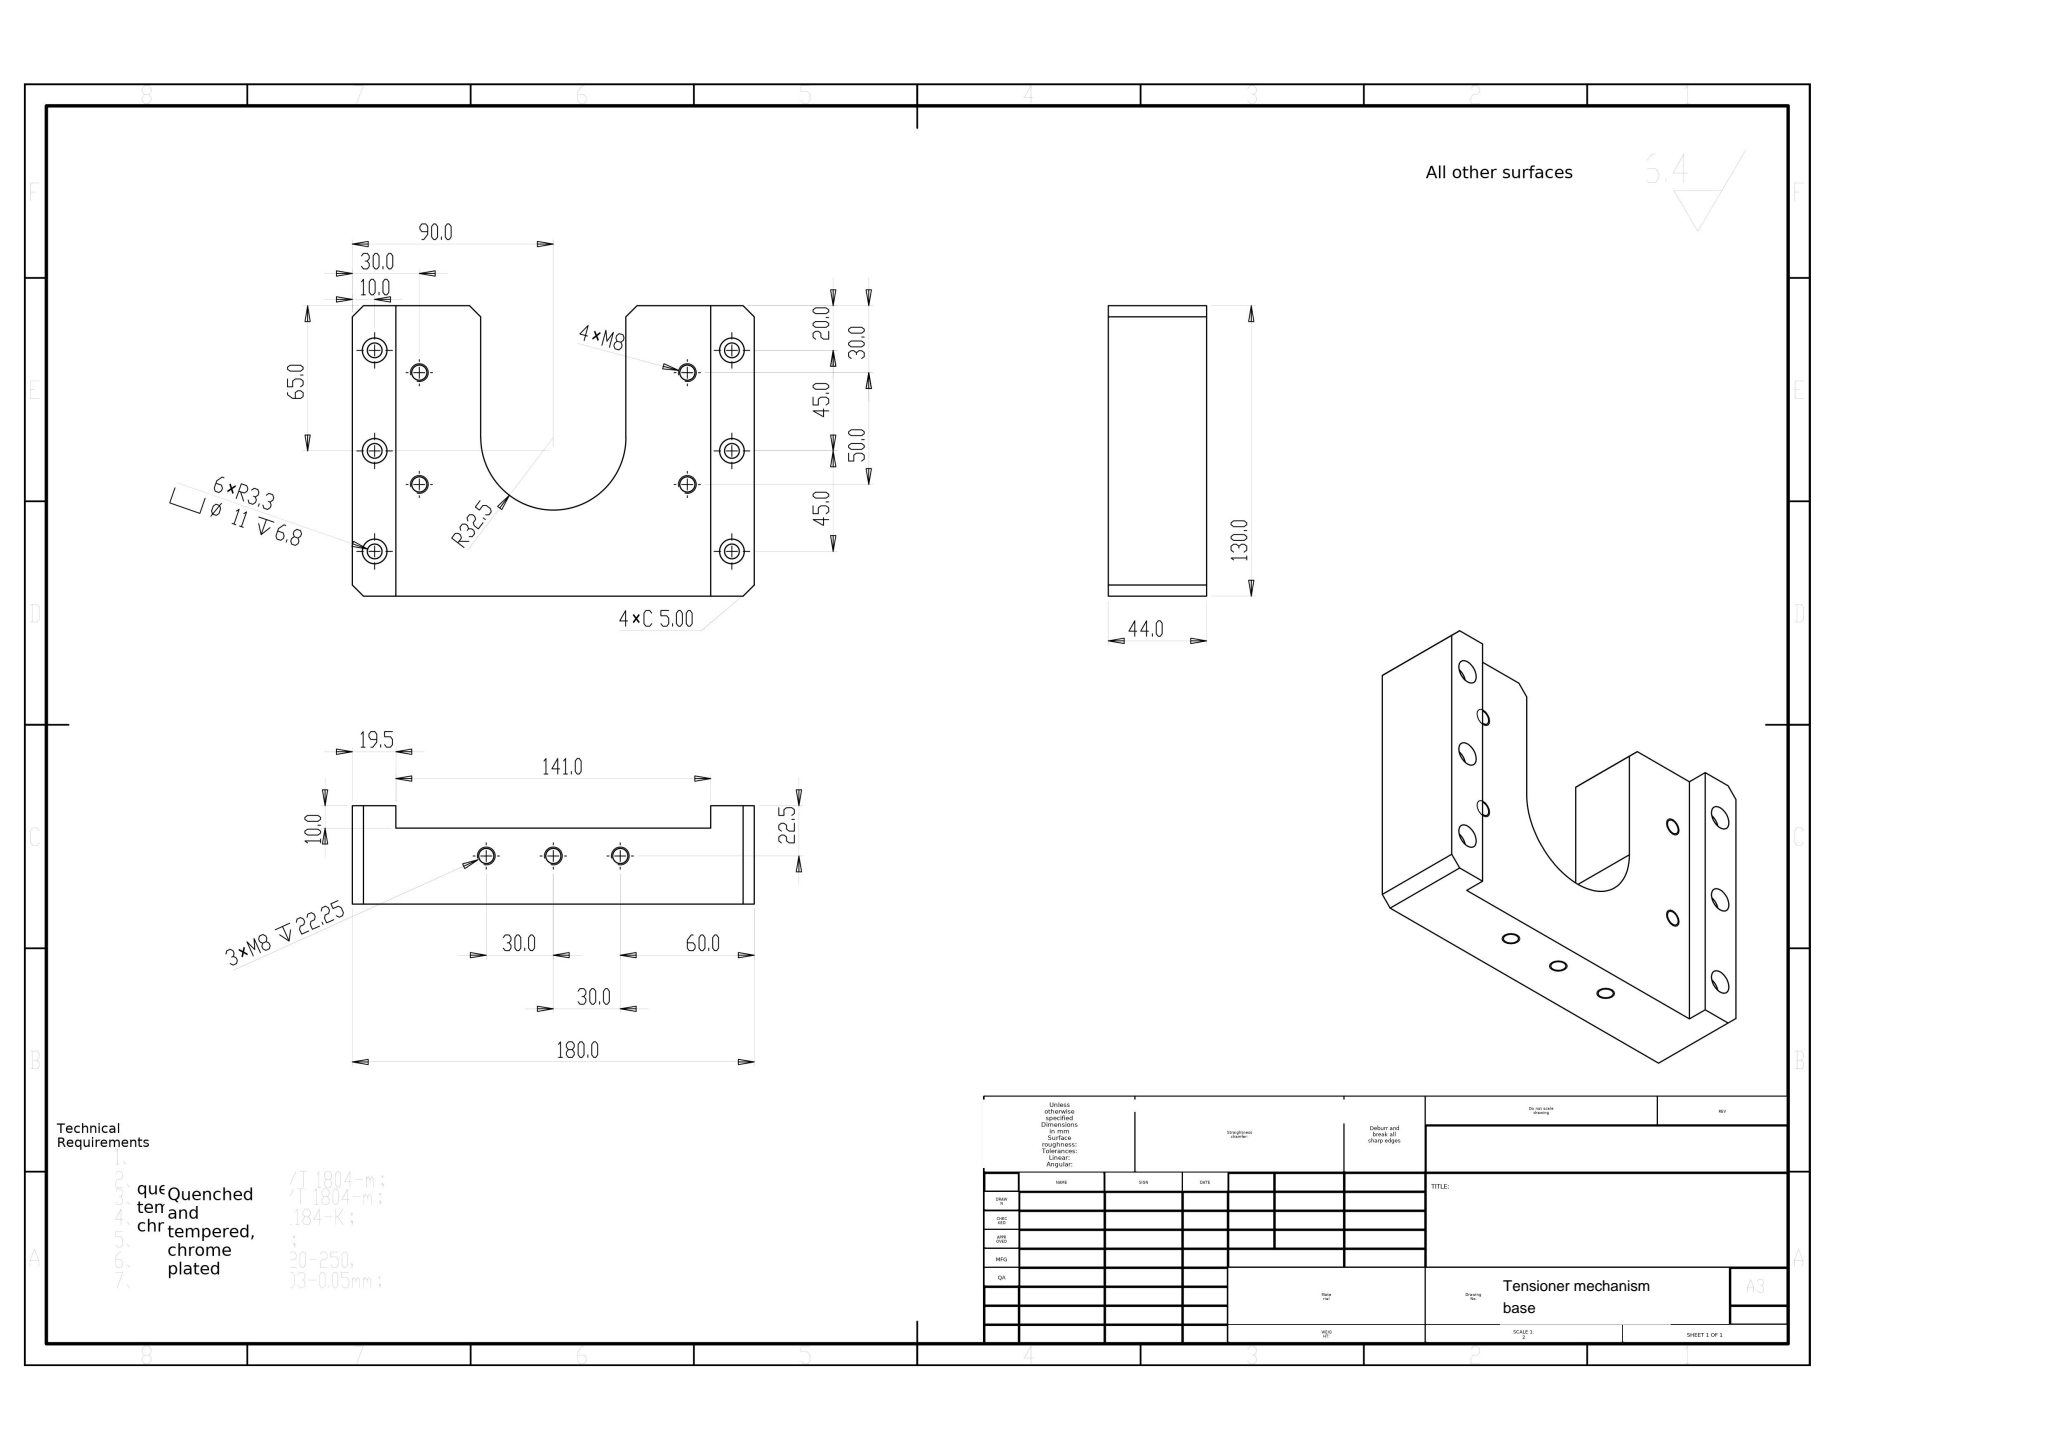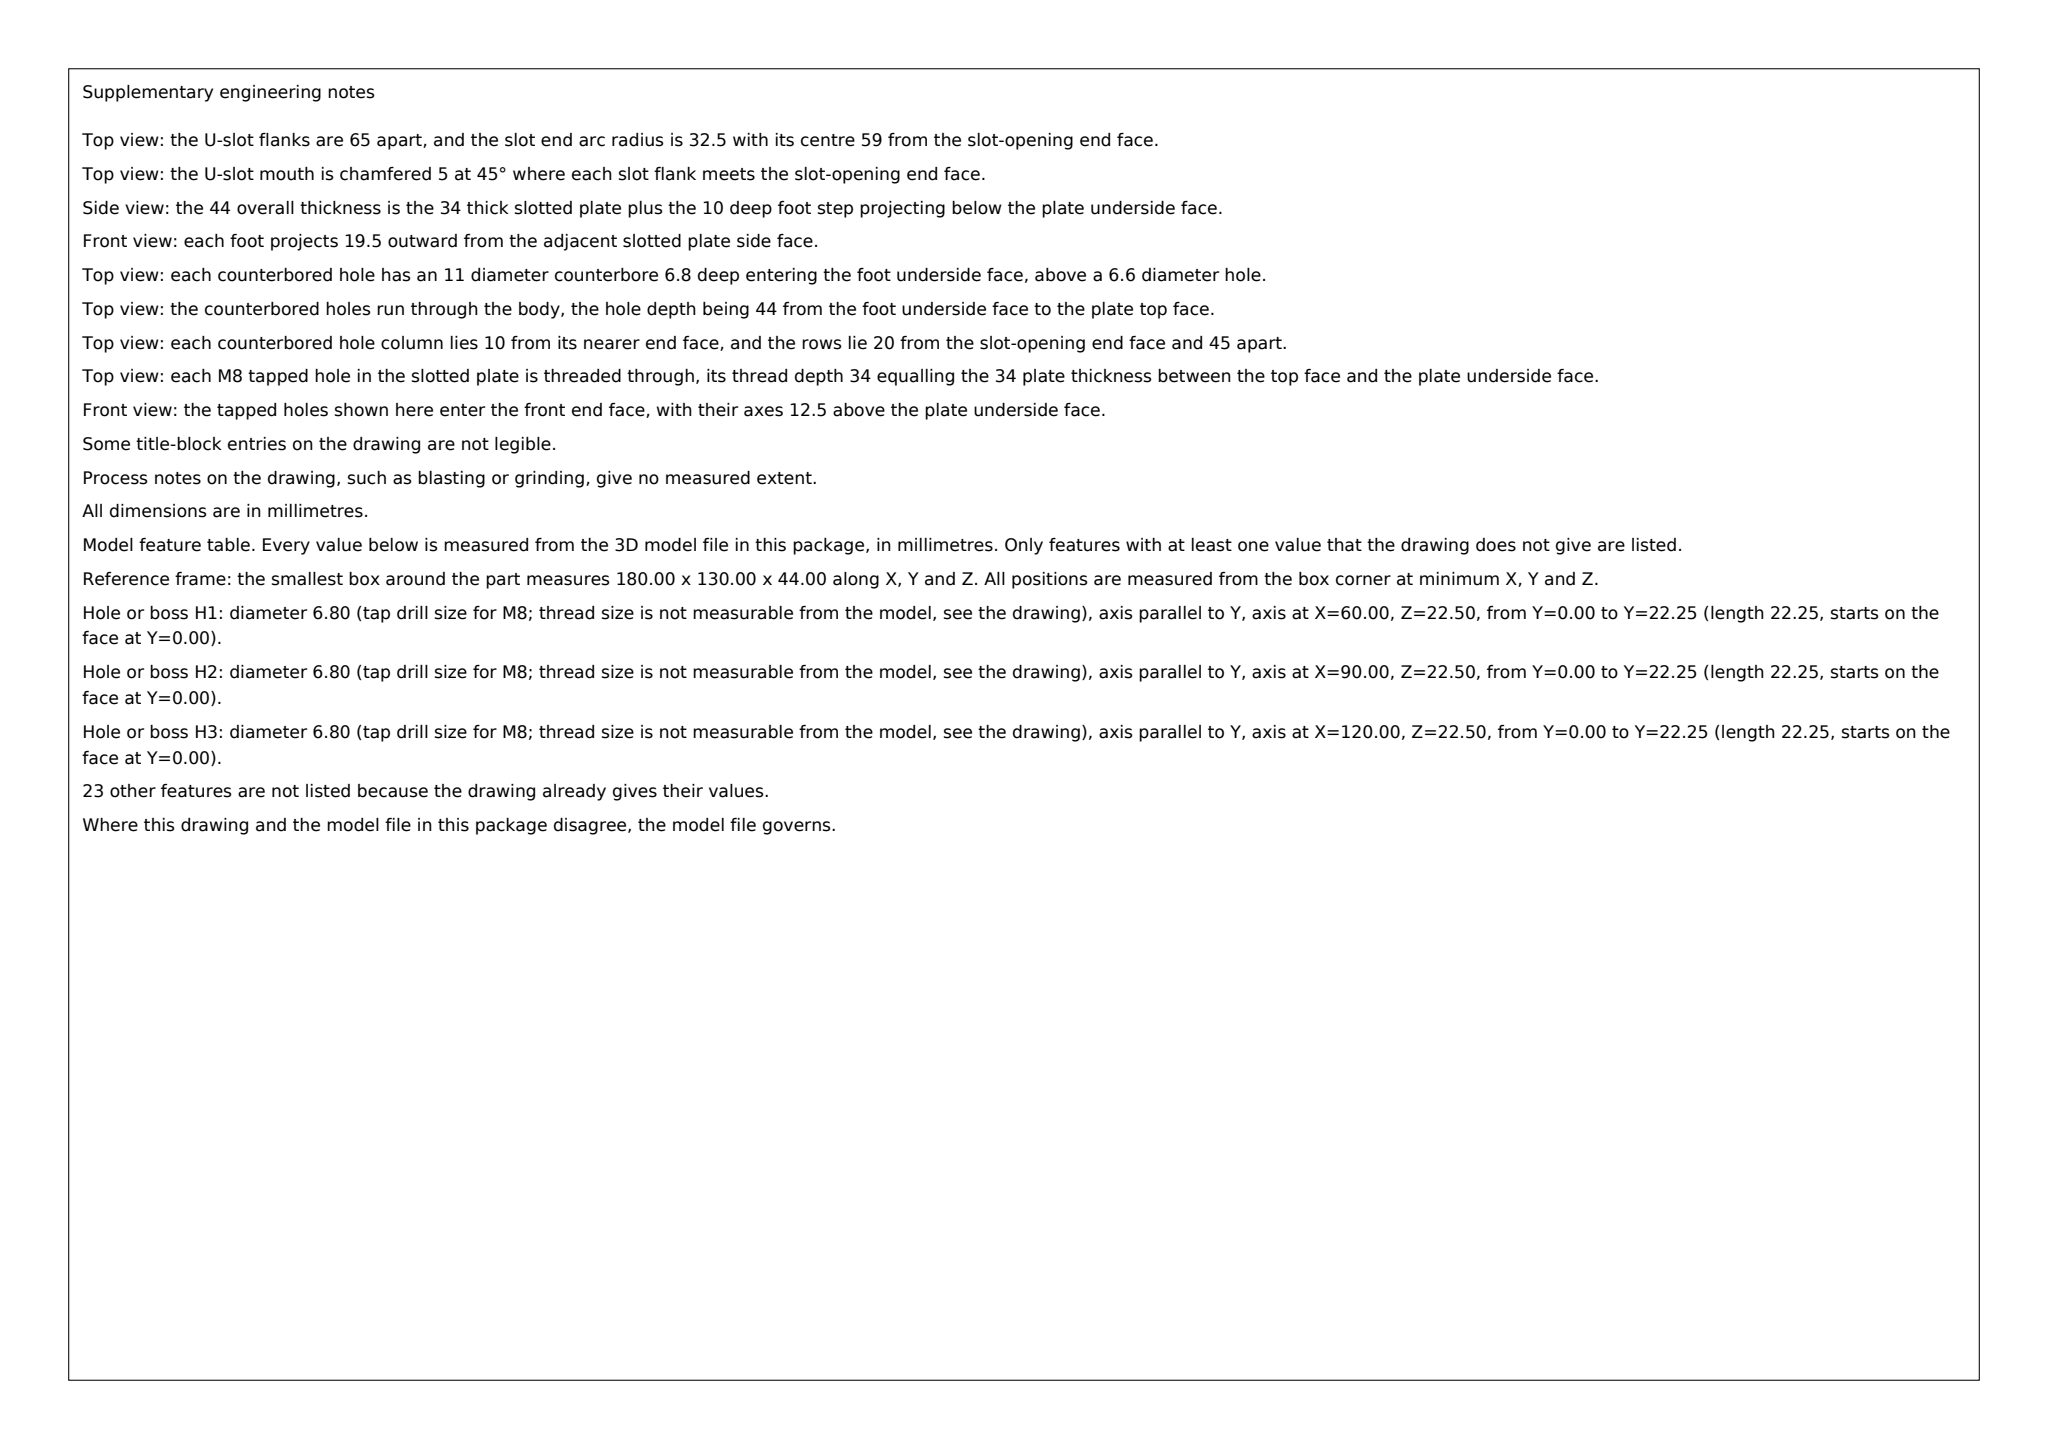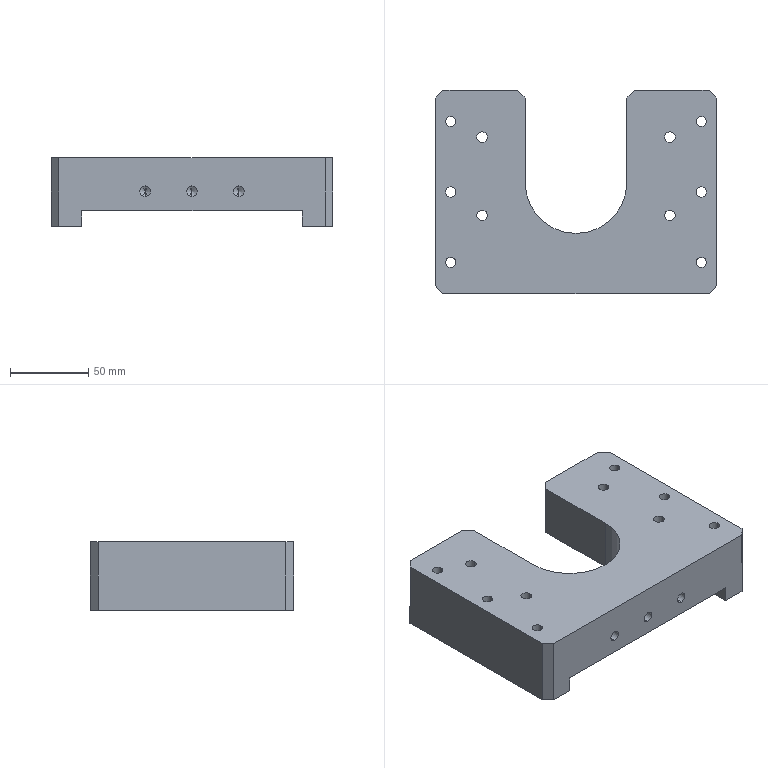Part | SolidWorks | mm | 1 solid | 70 faces | box 180 x 130 x 44 mm | volume 637498 mm3 | cylinder 39 | plane 25 | cone 6 | commonest cylinder face diameters 6.8 x14 11 x12 6.6 x12 65 x1
Drawing notes:
U-SLOT 65 WIDE x 91.5 DP FROM TOP, CL 90 FROM LEFT EDGE (R32.5) | from the solid: cyl Ø65 axis z at (90,71); side walls x=57.5/122.5; 130-(71-32.5)=91.5
6x Ø6.6 THRU, Ø11 CBORE DP 6.8; CL 10 FROM LEFT EDGE & 10 FROM RIGHT EDGE | from the solid: Ø6.6 thru + Ø11↧6.8 at x=10 and x=170, bbox X=180
4x M8 THREAD DP 33, DRILL Ø6.8 DP 34 BLIND FROM FRONT FACE | from the solid: Ø6.8 z-holes len 34 in 44 thk plate, 118° drill point cones ref Ø6.8
4x M8 CL AT 30 & 150 FROM LEFT EDGE | from the solid: Ø6.8 z-holes at (30,50),(30,100),(150,50),(150,100)
build123d program:
from build123d import *

# Parameters (mm, degrees)
SKETCH1_W                                            = 180
SKETCH1_H                                            = 130
BOSS_EXTRUDE1_DEPTH                                  = 34
M8_TAPPED_HOLE1_D                                    = 6.8
M8_TAPPED_HOLE1_DEPTH                                = 22.25
M8_TAPPED_HOLE1_TIP                                  = 2.043
SKETCH10_W                                           = 19.5
SKETCH10_H                                           = 130
BOSS_EXTRUDE2_DEPTH                                  = 10
HOLE_SIZE_ACCORDING_TO_THE_TYPE_OF_HEXAG_D           = 6.6
HOLE_SIZE_ACCORDING_TO_THE_TYPE_OF_HEXAG_CBORE_D     = 11
HOLE_SIZE_ACCORDING_TO_THE_TYPE_OF_HEXAG_CBORE_DEPTH = 6.8
CUT_EXTRUDE2_DEPTH                                   = 117.108
CHAMFER1_SIZE                                        = 5
M8_TAPPED_HOLE2_D                                    = 6.8


with BuildPart() as part:
    # Sketch1 → Boss-Extrude1 (new body)
    with BuildSketch(Plane.XY):
        Rectangle(SKETCH1_W, SKETCH1_H)
    extrude(amount=BOSS_EXTRUDE1_DEPTH)

    # M8 Tapped Hole1
    with Locations(Plane(origin=(0, -65, 0), x_dir=(-1, 0, 0), z_dir=(0, -1, 0))):
        with Locations((-30, -12.5), (0, -12.5), (30, -12.5)):
            Hole(M8_TAPPED_HOLE1_D / 2, depth=M8_TAPPED_HOLE1_DEPTH)
            with Locations((0, 0, -(M8_TAPPED_HOLE1_DEPTH + M8_TAPPED_HOLE1_TIP / 2))):  # 118° drill point
                Cone(0, M8_TAPPED_HOLE1_D / 2, M8_TAPPED_HOLE1_TIP, mode=Mode.SUBTRACT)

    # Sketch10 → Boss-Extrude2 (add)
    with BuildSketch(Plane(origin=(0, 0, 0), x_dir=(-1, 0, 0), z_dir=(0, 0, -1))):
        with Locations((-80.25, 0)):
            Rectangle(SKETCH10_W, SKETCH10_H)
    boss_extrude2 = extrude(amount=BOSS_EXTRUDE2_DEPTH)

    # Mirror3: Boss-Extrude2 across plane
    add(boss_extrude2.mirror(Plane(origin=(0, 0, 0), x_dir=(0, 0, 1), z_dir=(1, 0, 0))))

    # Hole size according to the type of hexag (through all)
    with Locations(Plane(origin=(6.354, -33.174, -10), x_dir=(-1, 0, 0), z_dir=(0, 0, -1))):
        with Locations((-73.646, 78.174), (-73.646, 33.174), (-73.646, -11.826)):
            hole_size_according_to_the_type_of_hexag = CounterBoreHole(HOLE_SIZE_ACCORDING_TO_THE_TYPE_OF_HEXAG_D / 2, HOLE_SIZE_ACCORDING_TO_THE_TYPE_OF_HEXAG_CBORE_D / 2, HOLE_SIZE_ACCORDING_TO_THE_TYPE_OF_HEXAG_CBORE_DEPTH)

    # Mirror2: Hole size according to the type of hexag across plane
    add(hole_size_according_to_the_type_of_hexag.mirror(Plane(origin=(0, 0, 0), x_dir=(0, 0, 1), z_dir=(1, 0, 0))), mode=Mode.SUBTRACT)

    # Sketch8 → Cut-Extrude2 (cut, through all)
    with BuildSketch(Plane(origin=(0, 0, 0), x_dir=(-1, 0, 0), z_dir=(0, 0, -1))):
        with BuildLine():
            Line((-32.5, 6), (-32.5, 82.983))
            Line((-32.5, 82.983), (32.5, 82.983))
            Line((32.5, 82.983), (32.5, 6))
            ThreePointArc((32.5, 6), (0, -26.5), (-32.5, 6))
        make_face()
    extrude(amount=-CUT_EXTRUDE2_DEPTH, mode=Mode.SUBTRACT)

    # Chamfer1
    chamfer1_edges = [part.edges().sort_by_distance(p)[0] for p in [
        (-32.5, 65, 17),
        (32.5, 65, 17),
        (90, 65, 12),
        (-90, 65, 12),
        (-90, -65, 12),
        (90, -65, 12),
    ]]
    chamfer(chamfer1_edges, length=CHAMFER1_SIZE)

    # M8 Tapped Hole2 (through all)
    with Locations(Plane(origin=(60, 35, 0), x_dir=(-1, 0, 0), z_dir=(0, 0, -1))):
        with Locations((0, 0), (0, -50), (120, -50), (120, 0)):
            Hole(M8_TAPPED_HOLE2_D / 2)


solid = part.part